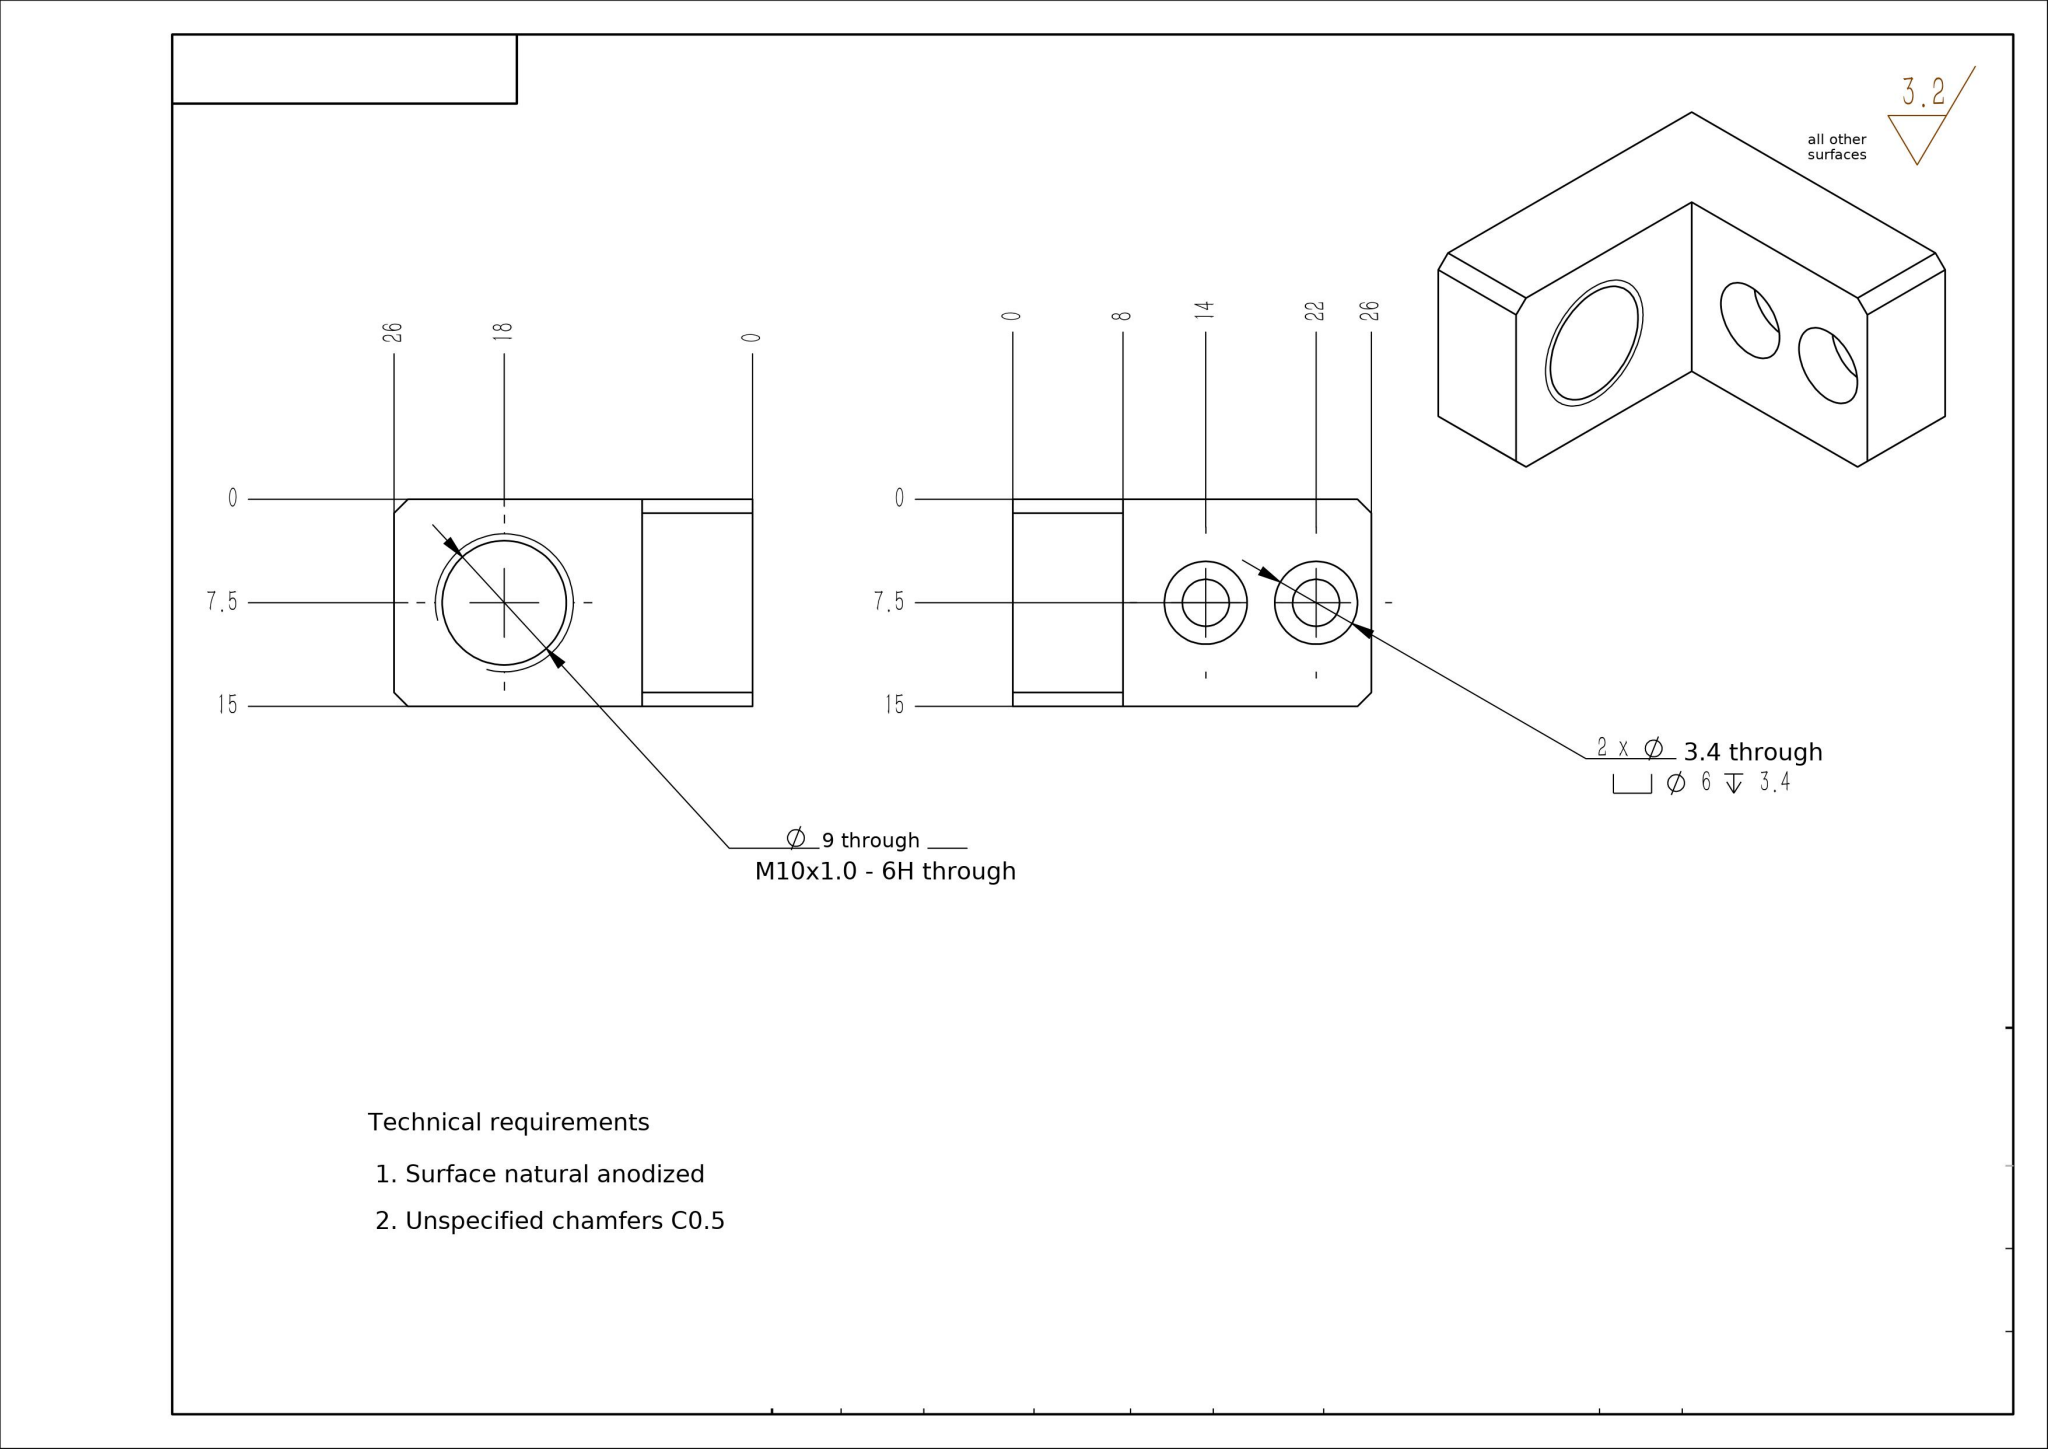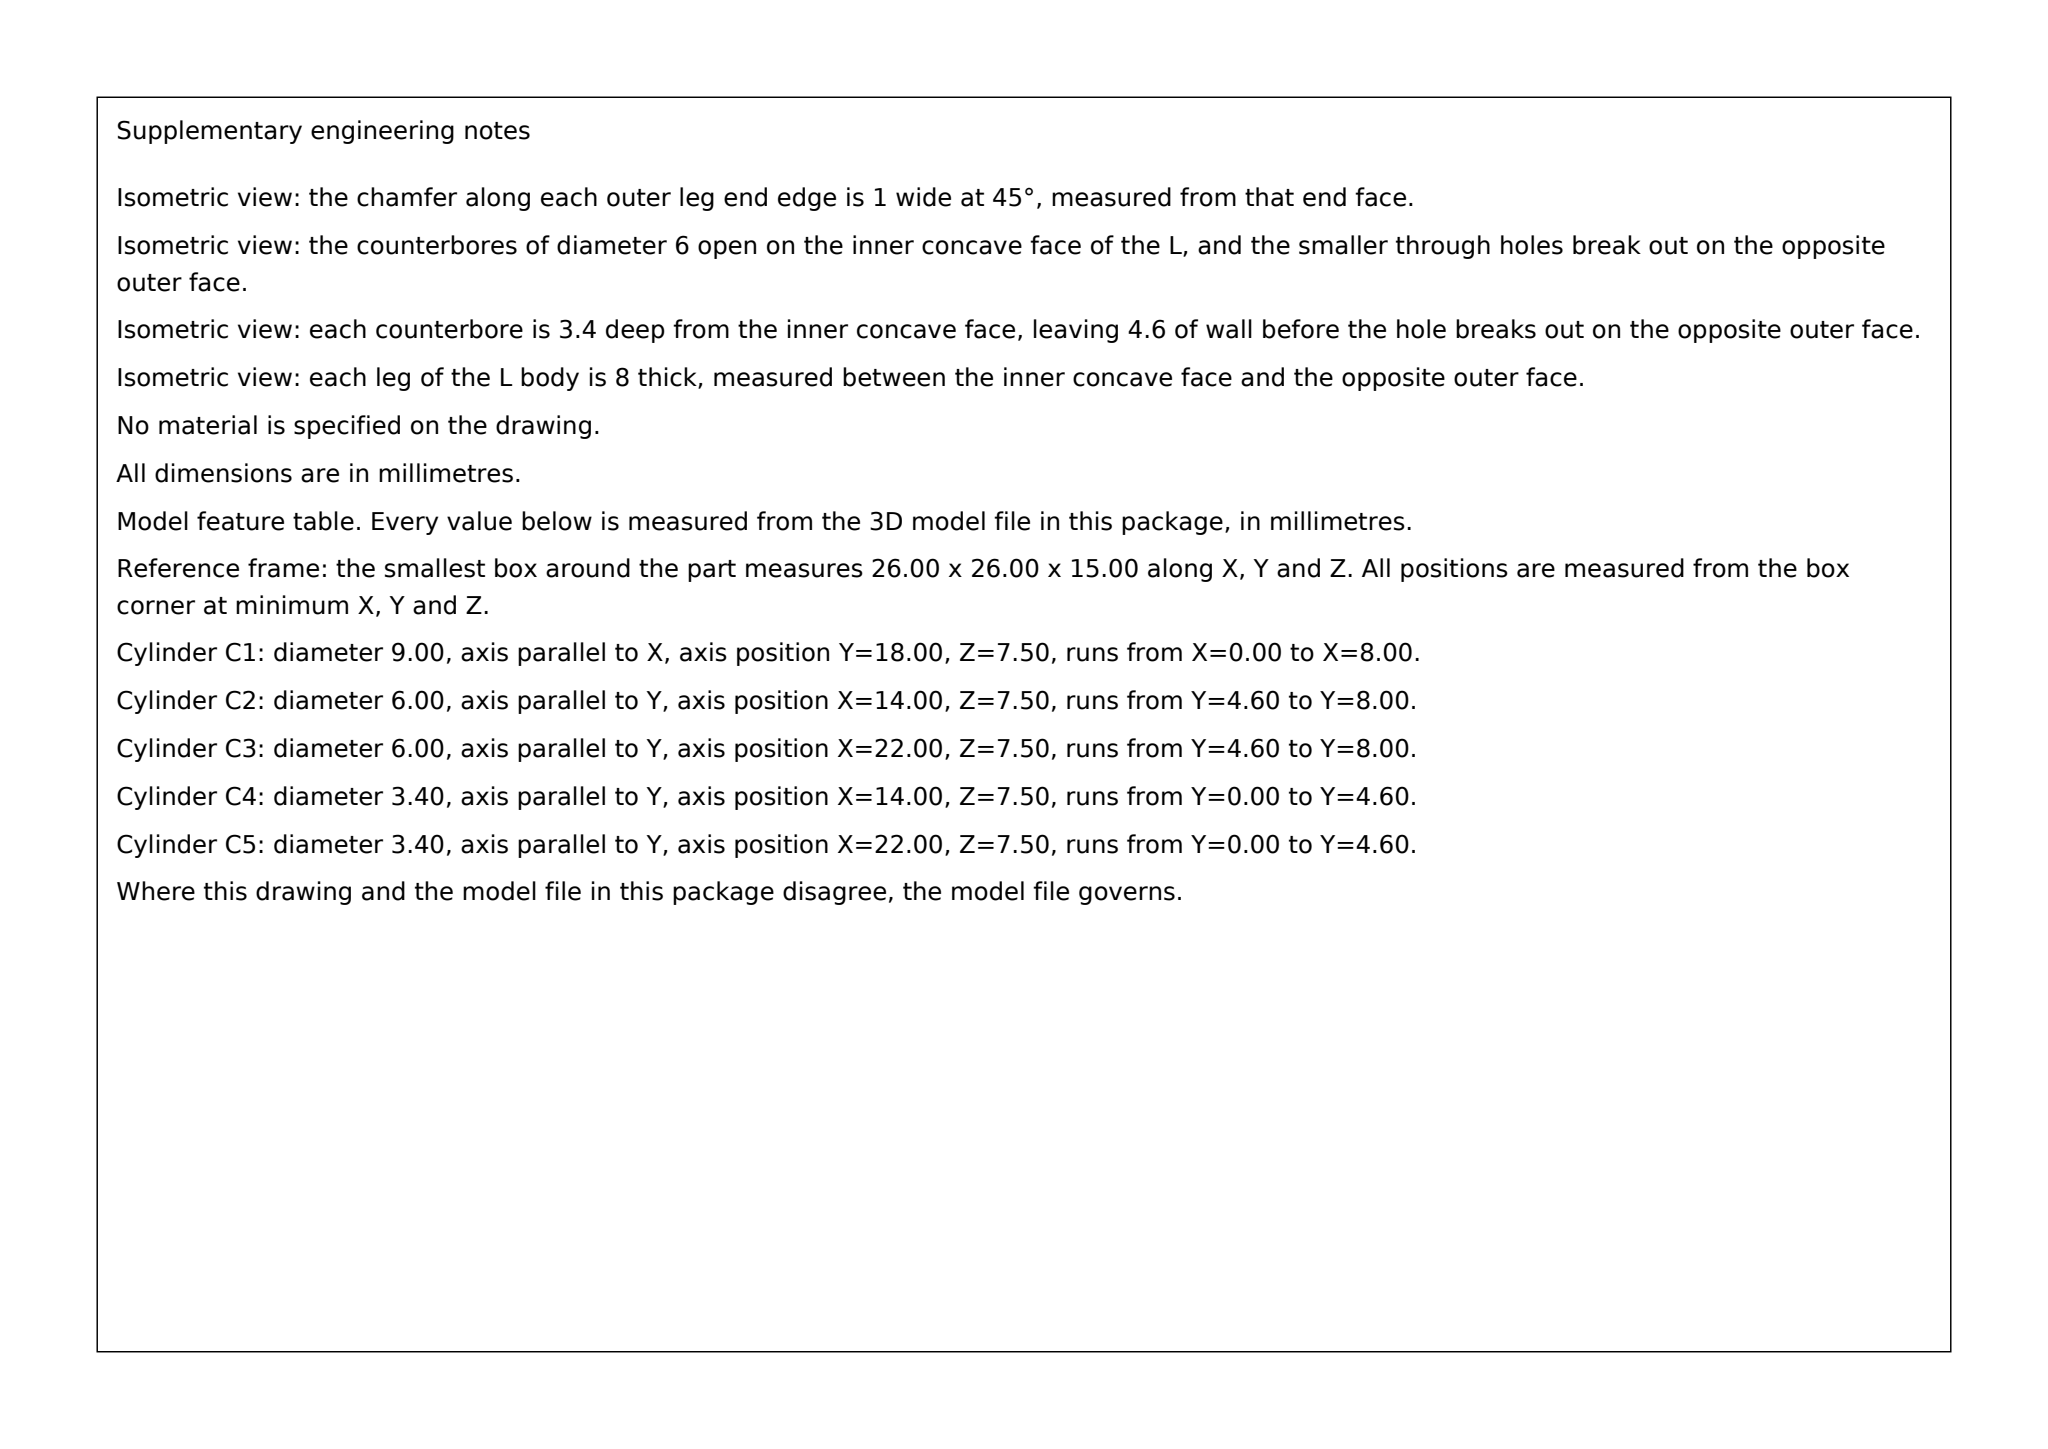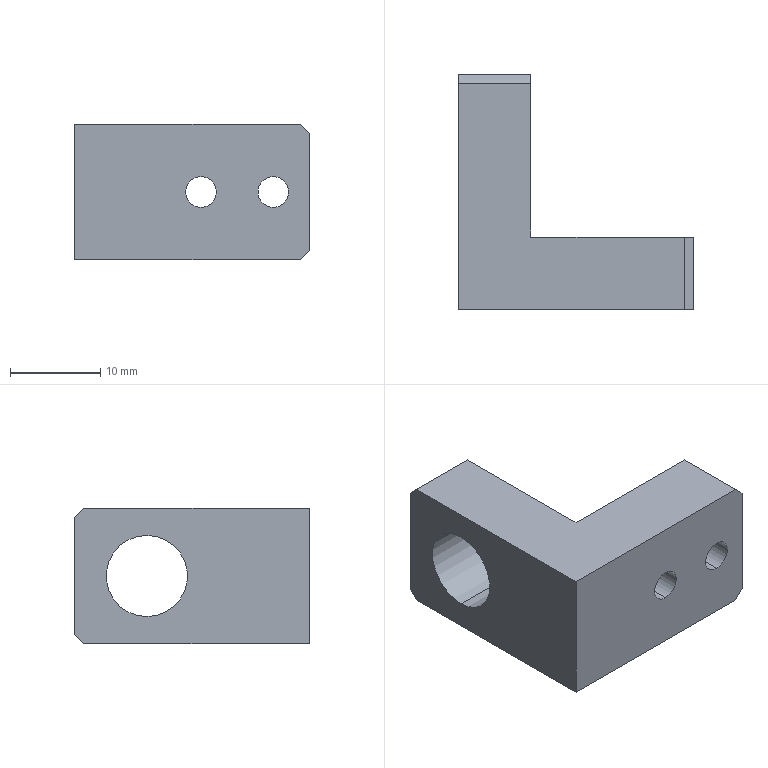Part | SolidWorks | mm | 1 solid | 24 faces | box 26 x 26 x 15 mm | volume 4479 mm3 | plane 14 | cylinder 10 | commonest cylinder face diameters 6 x4 3.4 x4 9 x2
Drawing notes:
LEG THK 8: STEP FACE AT ORD 8 FROM 0 DATUM, BOTH LEGS | from the solid: Planar face y=8 over x 8-26, z 0-15; face x=8 over y 8-26 (symmetric legs, bbox 26x26x15)
4X C1 x 45 ON OUTER CORNER EDGES, 8 LG (NOT C0.5) | from the solid: 4 inclined planes at 45 deg, size 1 x 8 x 1, at x=25/y=25 with z=0 and z=14
M10x1.0-6H THRU 8; Ø9 DRILL THRU | from the solid: Ø9 cylinder, axis x, at y=18 z=7.5, from x=0 to x=8 (full leg thk)
build123d program:
from build123d import *

# Parameters (mm, degrees)
BOSS_EXTRUDE1_DEPTH                               = 15
HOLE_SIZE_ACCORDING_TO_HEXAGON_SOCKET_D           = 3.4
HOLE_SIZE_ACCORDING_TO_HEXAGON_SOCKET_CBORE_D     = 6
HOLE_SIZE_ACCORDING_TO_HEXAGON_SOCKET_CBORE_DEPTH = 3.4
M10X1_0_TAPPED_HOLE1_D                            = 9
CHAMFER1_SIZE                                     = 1
CHAMFER2_SIZE                                     = 1


with BuildPart() as part:
    # Sketch1 → Boss-Extrude1 (new body)
    with BuildSketch(Plane.XY):
        Polygon((-13.935, 19.774), (-13.935, -6.226), (12.065, -6.226), (12.065, 1.774), (-5.935, 1.774), (-5.935, 19.774), align=None)
    extrude(amount=BOSS_EXTRUDE1_DEPTH)

    # Hole Size _ according to_ Hexagon Socket (through all)
    with Locations(Plane(origin=(0, 1.774, 0), x_dir=(1, 0, 0), z_dir=(0, 1, 0))):
        with Locations((8.065, -7.5), (0.06452, -7.5)):
            CounterBoreHole(HOLE_SIZE_ACCORDING_TO_HEXAGON_SOCKET_D / 2, HOLE_SIZE_ACCORDING_TO_HEXAGON_SOCKET_CBORE_D / 2, HOLE_SIZE_ACCORDING_TO_HEXAGON_SOCKET_CBORE_DEPTH)

    # M10x1.0 Tapped Hole1 (through all)
    with Locations(Plane(origin=(-5.935, 0, 0), x_dir=(0, 0, -1), z_dir=(1, 0, 0))):
        with Locations((-7.5, 11.774)):
            Hole(M10X1_0_TAPPED_HOLE1_D / 2)

    # Chamfer1
    chamfer1_edges = [part.edges().sort_by_distance(p)[0] for p in [
        (12.065, -2.226, 15),
        (12.065, -2.226, 0),
    ]]
    chamfer(chamfer1_edges, length=CHAMFER1_SIZE)

    # Chamfer2
    chamfer2_edges = [part.edges().sort_by_distance(p)[0] for p in [
        (-9.935, 19.774, 15),
        (-9.935, 19.774, 0),
    ]]
    chamfer(chamfer2_edges, length=CHAMFER2_SIZE)


solid = part.part
STEP:
#1=CARTESIAN_POINT('',(-13.935,11.774,12.));
#2=VERTEX_POINT('',#1);
#3=CARTESIAN_POINT('',(-13.935,11.774,3.));
#4=VERTEX_POINT('',#3);
#5=CARTESIAN_POINT('',(-13.935,11.774,7.5));
#6=DIRECTION('',(1.,0.,0.));
#7=DIRECTION('',(0.,0.,-1.));
#8=AXIS2_PLACEMENT_3D('',#5,#6,#7);
#9=CIRCLE('',#8,4.5);
#10=EDGE_CURVE('',#2,#4,#9,.T.);
#11=ORIENTED_EDGE('',*,*,#10,.F.);
#12=CARTESIAN_POINT('',(-5.935,11.774,12.));
#13=VERTEX_POINT('',#12);
#14=CARTESIAN_POINT('',(-5.935,11.774,12.));
#15=DIRECTION('',(1.,0.,0.));
#16=VECTOR('',#15,1000.);
#17=LINE('',#14,#16);
#18=EDGE_CURVE('',#2,#13,#17,.T.);
#19=ORIENTED_EDGE('',*,*,#18,.T.);
#20=CARTESIAN_POINT('',(-5.935,11.774,3.));
#21=VERTEX_POINT('',#20);
#22=CARTESIAN_POINT('',(-5.935,11.774,7.5));
#23=DIRECTION('',(1.,0.,0.));
#24=DIRECTION('',(0.,0.,-1.));
#25=AXIS2_PLACEMENT_3D('',#22,#23,#24);
#26=CIRCLE('',#25,4.5);
#27=EDGE_CURVE('',#13,#21,#26,.T.);
#28=ORIENTED_EDGE('',*,*,#27,.T.);
#29=CARTESIAN_POINT('',(-5.935,11.774,3.));
#30=DIRECTION('',(1.,0.,0.));
#31=VECTOR('',#30,1000.);
#32=LINE('',#29,#31);
#33=EDGE_CURVE('',#4,#21,#32,.T.);
#34=ORIENTED_EDGE('',*,*,#33,.F.);
#35=EDGE_LOOP('',(#11,#19,#28,#34));
#36=FACE_OUTER_BOUND('',#35,.T.);
#37=CARTESIAN_POINT('',(-5.935,11.774,7.5));
#38=DIRECTION('',(1.,0.,0.));
#39=DIRECTION('',(0.,0.,-1.));
#40=AXIS2_PLACEMENT_3D('',#37,#38,#39);
#41=CYLINDRICAL_SURFACE('',#40,4.5);
#42=ADVANCED_FACE('',(#36),#41,.F.);
#43=CARTESIAN_POINT('',(8.065,-1.626,4.5));
#44=VERTEX_POINT('',#43);
#45=CARTESIAN_POINT('',(8.065,-1.626,10.5));
#46=VERTEX_POINT('',#45);
#47=CARTESIAN_POINT('',(8.065,-1.626,7.5));
#48=DIRECTION('',(0.,1.,0.));
#49=DIRECTION('',(0.,0.,1.));
#50=AXIS2_PLACEMENT_3D('',#47,#48,#49);
#51=CIRCLE('',#50,3.);
#52=EDGE_CURVE('',#44,#46,#51,.T.);
#53=ORIENTED_EDGE('',*,*,#52,.F.);
#54=CARTESIAN_POINT('',(8.065,1.774,4.5));
#55=VERTEX_POINT('',#54);
#56=CARTESIAN_POINT('',(8.065,1.774,4.5));
#57=DIRECTION('',(0.,1.,0.));
#58=VECTOR('',#57,1000.);
#59=LINE('',#56,#58);
#60=EDGE_CURVE('',#44,#55,#59,.T.);
#61=ORIENTED_EDGE('',*,*,#60,.T.);
#62=CARTESIAN_POINT('',(8.065,1.774,10.5));
#63=VERTEX_POINT('',#62);
#64=CARTESIAN_POINT('',(8.065,1.774,7.5));
#65=DIRECTION('',(0.,1.,0.));
#66=DIRECTION('',(0.,0.,1.));
#67=AXIS2_PLACEMENT_3D('',#64,#65,#66);
#68=CIRCLE('',#67,3.);
#69=EDGE_CURVE('',#55,#63,#68,.T.);
#70=ORIENTED_EDGE('',*,*,#69,.T.);
#71=CARTESIAN_POINT('',(8.065,1.774,10.5));
#72=DIRECTION('',(0.,1.,0.));
#73=VECTOR('',#72,1000.);
#74=LINE('',#71,#73);
#75=EDGE_CURVE('',#46,#63,#74,.T.);
#76=ORIENTED_EDGE('',*,*,#75,.F.);
#77=EDGE_LOOP('',(#53,#61,#70,#76));
#78=FACE_OUTER_BOUND('',#77,.T.);
#79=CARTESIAN_POINT('',(8.065,1.774,7.5));
#80=DIRECTION('',(0.,1.,0.));
#81=DIRECTION('',(0.,0.,1.));
#82=AXIS2_PLACEMENT_3D('',#79,#80,#81);
#83=CYLINDRICAL_SURFACE('',#82,3.);
#84=ADVANCED_FACE('',(#78),#83,.F.);
#85=CARTESIAN_POINT('',(8.065,-6.226,5.8));
#86=VERTEX_POINT('',#85);
#87=CARTESIAN_POINT('',(8.065,-6.226,9.2));
#88=VERTEX_POINT('',#87);
#89=CARTESIAN_POINT('',(8.065,-6.226,7.5));
#90=DIRECTION('',(0.,1.,0.));
#91=DIRECTION('',(0.,0.,1.));
#92=AXIS2_PLACEMENT_3D('',#89,#90,#91);
#93=CIRCLE('',#92,1.7);
#94=EDGE_CURVE('',#86,#88,#93,.T.);
#95=ORIENTED_EDGE('',*,*,#94,.F.);
#96=CARTESIAN_POINT('',(8.065,-1.626,5.8));
#97=VERTEX_POINT('',#96);
#98=CARTESIAN_POINT('',(8.065,1.774,5.8));
#99=DIRECTION('',(0.,1.,0.));
#100=VECTOR('',#99,1000.);
#101=LINE('',#98,#100);
#102=EDGE_CURVE('',#86,#97,#101,.T.);
#103=ORIENTED_EDGE('',*,*,#102,.T.);
#104=CARTESIAN_POINT('',(8.065,-1.626,9.2));
#105=VERTEX_POINT('',#104);
#106=CARTESIAN_POINT('',(8.065,-1.626,7.5));
#107=DIRECTION('',(0.,1.,0.));
#108=DIRECTION('',(0.,0.,1.));
#109=AXIS2_PLACEMENT_3D('',#106,#107,#108);
#110=CIRCLE('',#109,1.7);
#111=EDGE_CURVE('',#97,#105,#110,.T.);
#112=ORIENTED_EDGE('',*,*,#111,.T.);
#113=CARTESIAN_POINT('',(8.065,1.774,9.2));
#114=DIRECTION('',(0.,1.,0.));
#115=VECTOR('',#114,1000.);
#116=LINE('',#113,#115);
#117=EDGE_CURVE('',#88,#105,#116,.T.);
#118=ORIENTED_EDGE('',*,*,#117,.F.);
#119=EDGE_LOOP('',(#95,#103,#112,#118));
#120=FACE_OUTER_BOUND('',#119,.T.);
#121=CARTESIAN_POINT('',(8.065,1.774,7.5));
#122=DIRECTION('',(0.,1.,0.));
#123=DIRECTION('',(0.,0.,1.));
#124=AXIS2_PLACEMENT_3D('',#121,#122,#123);
#125=CYLINDRICAL_SURFACE('',#124,1.7);
#126=ADVANCED_FACE('',(#120),#125,.F.);
#127=CARTESIAN_POINT('',(0.06452,-1.626,4.5));
#128=VERTEX_POINT('',#127);
#129=CARTESIAN_POINT('',(0.06452,-1.626,10.5));
#130=VERTEX_POINT('',#129);
#131=CARTESIAN_POINT('',(0.06452,-1.626,7.5));
#132=DIRECTION('',(0.,1.,0.));
#133=DIRECTION('',(0.,0.,1.));
#134=AXIS2_PLACEMENT_3D('',#131,#132,#133);
#135=CIRCLE('',#134,3.);
#136=EDGE_CURVE('',#128,#130,#135,.T.);
#137=ORIENTED_EDGE('',*,*,#136,.F.);
#138=CARTESIAN_POINT('',(0.06452,1.774,4.5));
#139=VERTEX_POINT('',#138);
#140=CARTESIAN_POINT('',(0.06452,1.774,4.5));
#141=DIRECTION('',(0.,1.,0.));
#142=VECTOR('',#141,1000.);
#143=LINE('',#140,#142);
#144=EDGE_CURVE('',#128,#139,#143,.T.);
#145=ORIENTED_EDGE('',*,*,#144,.T.);
#146=CARTESIAN_POINT('',(0.06452,1.774,10.5));
#147=VERTEX_POINT('',#146);
#148=CARTESIAN_POINT('',(0.06452,1.774,7.5));
#149=DIRECTION('',(0.,1.,0.));
#150=DIRECTION('',(0.,0.,1.));
#151=AXIS2_PLACEMENT_3D('',#148,#149,#150);
#152=CIRCLE('',#151,3.);
#153=EDGE_CURVE('',#139,#147,#152,.T.);
#154=ORIENTED_EDGE('',*,*,#153,.T.);
#155=CARTESIAN_POINT('',(0.06452,1.774,10.5));
#156=DIRECTION('',(0.,1.,0.));
#157=VECTOR('',#156,1000.);
#158=LINE('',#155,#157);
#159=EDGE_CURVE('',#130,#147,#158,.T.);
#160=ORIENTED_EDGE('',*,*,#159,.F.);
#161=EDGE_LOOP('',(#137,#145,#154,#160));
#162=FACE_OUTER_BOUND('',#161,.T.);
#163=CARTESIAN_POINT('',(0.06452,1.774,7.5));
#164=DIRECTION('',(0.,1.,0.));
#165=DIRECTION('',(0.,0.,1.));
#166=AXIS2_PLACEMENT_3D('',#163,#164,#165);
#167=CYLINDRICAL_SURFACE('',#166,3.);
#168=ADVANCED_FACE('',(#162),#167,.F.);
#169=CARTESIAN_POINT('',(0.06452,-6.226,5.8));
#170=VERTEX_POINT('',#169);
#171=CARTESIAN_POINT('',(0.06452,-6.226,9.2));
#172=VERTEX_POINT('',#171);
#173=CARTESIAN_POINT('',(0.06452,-6.226,7.5));
#174=DIRECTION('',(0.,1.,0.));
#175=DIRECTION('',(0.,0.,1.));
#176=AXIS2_PLACEMENT_3D('',#173,#174,#175);
#177=CIRCLE('',#176,1.7);
#178=EDGE_CURVE('',#170,#172,#177,.T.);
#179=ORIENTED_EDGE('',*,*,#178,.F.);
#180=CARTESIAN_POINT('',(0.06452,-1.626,5.8));
#181=VERTEX_POINT('',#180);
#182=CARTESIAN_POINT('',(0.06452,1.774,5.8));
#183=DIRECTION('',(0.,1.,0.));
#184=VECTOR('',#183,1000.);
#185=LINE('',#182,#184);
#186=EDGE_CURVE('',#170,#181,#185,.T.);
#187=ORIENTED_EDGE('',*,*,#186,.T.);
#188=CARTESIAN_POINT('',(0.06452,-1.626,9.2));
#189=VERTEX_POINT('',#188);
#190=CARTESIAN_POINT('',(0.06452,-1.626,7.5));
#191=DIRECTION('',(0.,1.,0.));
#192=DIRECTION('',(0.,0.,1.));
#193=AXIS2_PLACEMENT_3D('',#190,#191,#192);
#194=CIRCLE('',#193,1.7);
#195=EDGE_CURVE('',#181,#189,#194,.T.);
#196=ORIENTED_EDGE('',*,*,#195,.T.);
#197=CARTESIAN_POINT('',(0.06452,1.774,9.2));
#198=DIRECTION('',(0.,1.,0.));
#199=VECTOR('',#198,1000.);
#200=LINE('',#197,#199);
#201=EDGE_CURVE('',#172,#189,#200,.T.);
#202=ORIENTED_EDGE('',*,*,#201,.F.);
#203=EDGE_LOOP('',(#179,#187,#196,#202));
#204=FACE_OUTER_BOUND('',#203,.T.);
#205=CARTESIAN_POINT('',(0.06452,1.774,7.5));
#206=DIRECTION('',(0.,1.,0.));
#207=DIRECTION('',(0.,0.,1.));
#208=AXIS2_PLACEMENT_3D('',#205,#206,#207);
#209=CYLINDRICAL_SURFACE('',#208,1.7);
#210=ADVANCED_FACE('',(#204),#209,.F.);
#211=CARTESIAN_POINT('',(-5.935,19.774,14.));
#212=VERTEX_POINT('',#211);
#213=CARTESIAN_POINT('',(-5.935,19.774,1.));
#214=VERTEX_POINT('',#213);
#215=CARTESIAN_POINT('',(-5.935,19.774,15.));
#216=DIRECTION('',(0.,0.,-1.));
#217=VECTOR('',#216,1000.);
#218=LINE('',#215,#217);
#219=EDGE_CURVE('',#212,#214,#218,.T.);
#220=ORIENTED_EDGE('',*,*,#219,.T.);
#221=CARTESIAN_POINT('',(-13.935,19.774,1.));
#222=VERTEX_POINT('',#221);
#223=CARTESIAN_POINT('',(-5.935,19.774,1.));
#224=DIRECTION('',(-1.,0.,0.));
#225=VECTOR('',#224,1000.);
#226=LINE('',#223,#225);
#227=EDGE_CURVE('',#214,#222,#226,.T.);
#228=ORIENTED_EDGE('',*,*,#227,.T.);
#229=CARTESIAN_POINT('',(-13.935,19.774,14.));
#230=VERTEX_POINT('',#229);
#231=CARTESIAN_POINT('',(-13.935,19.774,15.));
#232=DIRECTION('',(0.,0.,-1.));
#233=VECTOR('',#232,1000.);
#234=LINE('',#231,#233);
#235=EDGE_CURVE('',#230,#222,#234,.T.);
#236=ORIENTED_EDGE('',*,*,#235,.F.);
#237=CARTESIAN_POINT('',(-5.935,19.774,14.));
#238=DIRECTION('',(1.,0.,0.));
#239=VECTOR('',#238,1000.);
#240=LINE('',#237,#239);
#241=EDGE_CURVE('',#230,#212,#240,.T.);
#242=ORIENTED_EDGE('',*,*,#241,.T.);
#243=EDGE_LOOP('',(#220,#228,#236,#242));
#244=FACE_OUTER_BOUND('',#243,.T.);
#245=CARTESIAN_POINT('',(-5.935,19.774,15.));
#246=DIRECTION('',(0.,-1.,0.));
#247=DIRECTION('',(0.,0.,-1.));
#248=AXIS2_PLACEMENT_3D('',#245,#246,#247);
#249=PLANE('',#248);
#250=ADVANCED_FACE('',(#244),#249,.F.);
#251=CARTESIAN_POINT('',(-13.935,11.774,7.5));
#252=DIRECTION('',(1.,0.,0.));
#253=DIRECTION('',(0.,0.,-1.));
#254=AXIS2_PLACEMENT_3D('',#251,#252,#253);
#255=CIRCLE('',#254,4.5);
#256=EDGE_CURVE('',#4,#2,#255,.T.);
#257=ORIENTED_EDGE('',*,*,#256,.T.);
#258=ORIENTED_EDGE('',*,*,#10,.T.);
#259=EDGE_LOOP('',(#257,#258));
#260=FACE_BOUND('',#259,.T.);
#261=ORIENTED_EDGE('',*,*,#235,.T.);
#262=CARTESIAN_POINT('',(-13.935,18.774,0.));
#263=VERTEX_POINT('',#262);
#264=CARTESIAN_POINT('',(-13.935,19.774,1.));
#265=DIRECTION('',(0.,-0.7071,-0.7071));
#266=VECTOR('',#265,1000.);
#267=LINE('',#264,#266);
#268=EDGE_CURVE('',#222,#263,#267,.T.);
#269=ORIENTED_EDGE('',*,*,#268,.T.);
#270=CARTESIAN_POINT('',(-13.935,-6.226,0.));
#271=VERTEX_POINT('',#270);
#272=CARTESIAN_POINT('',(-13.935,19.774,0.));
#273=DIRECTION('',(0.,-1.,0.));
#274=VECTOR('',#273,1000.);
#275=LINE('',#272,#274);
#276=EDGE_CURVE('',#263,#271,#275,.T.);
#277=ORIENTED_EDGE('',*,*,#276,.T.);
#278=CARTESIAN_POINT('',(-13.935,-6.226,15.));
#279=VERTEX_POINT('',#278);
#280=CARTESIAN_POINT('',(-13.935,-6.226,15.));
#281=DIRECTION('',(0.,0.,-1.));
#282=VECTOR('',#281,1000.);
#283=LINE('',#280,#282);
#284=EDGE_CURVE('',#279,#271,#283,.T.);
#285=ORIENTED_EDGE('',*,*,#284,.F.);
#286=CARTESIAN_POINT('',(-13.935,18.774,15.));
#287=VERTEX_POINT('',#286);
#288=CARTESIAN_POINT('',(-13.935,19.774,15.));
#289=DIRECTION('',(0.,-1.,0.));
#290=VECTOR('',#289,1000.);
#291=LINE('',#288,#290);
#292=EDGE_CURVE('',#287,#279,#291,.T.);
#293=ORIENTED_EDGE('',*,*,#292,.F.);
#294=CARTESIAN_POINT('',(-13.935,18.774,15.));
#295=DIRECTION('',(-0.,0.7071,-0.7071));
#296=VECTOR('',#295,1000.);
#297=LINE('',#294,#296);
#298=EDGE_CURVE('',#287,#230,#297,.T.);
#299=ORIENTED_EDGE('',*,*,#298,.T.);
#300=EDGE_LOOP('',(#261,#269,#277,#285,#293,#299));
#301=FACE_OUTER_BOUND('',#300,.T.);
#302=CARTESIAN_POINT('',(-13.935,19.774,15.));
#303=DIRECTION('',(1.,0.,0.));
#304=DIRECTION('',(-0.,1.,0.));
#305=AXIS2_PLACEMENT_3D('',#302,#303,#304);
#306=PLANE('',#305);
#307=ADVANCED_FACE('',(#260,#301),#306,.F.);
#308=CARTESIAN_POINT('',(8.065,-6.226,7.5));
#309=DIRECTION('',(0.,1.,0.));
#310=DIRECTION('',(0.,0.,1.));
#311=AXIS2_PLACEMENT_3D('',#308,#309,#310);
#312=CIRCLE('',#311,1.7);
#313=EDGE_CURVE('',#88,#86,#312,.T.);
#314=ORIENTED_EDGE('',*,*,#313,.T.);
#315=ORIENTED_EDGE('',*,*,#94,.T.);
#316=EDGE_LOOP('',(#314,#315));
#317=FACE_BOUND('',#316,.T.);
#318=CARTESIAN_POINT('',(0.06452,-6.226,7.5));
#319=DIRECTION('',(0.,1.,0.));
#320=DIRECTION('',(0.,0.,1.));
#321=AXIS2_PLACEMENT_3D('',#318,#319,#320);
#322=CIRCLE('',#321,1.7);
#323=EDGE_CURVE('',#172,#170,#322,.T.);
#324=ORIENTED_EDGE('',*,*,#323,.T.);
#325=ORIENTED_EDGE('',*,*,#178,.T.);
#326=EDGE_LOOP('',(#324,#325));
#327=FACE_BOUND('',#326,.T.);
#328=CARTESIAN_POINT('',(12.065,-6.226,14.));
#329=VERTEX_POINT('',#328);
#330=CARTESIAN_POINT('',(12.065,-6.226,1.));
#331=VERTEX_POINT('',#330);
#332=CARTESIAN_POINT('',(12.065,-6.226,15.));
#333=DIRECTION('',(0.,0.,-1.));
#334=VECTOR('',#333,1000.);
#335=LINE('',#332,#334);
#336=EDGE_CURVE('',#329,#331,#335,.T.);
#337=ORIENTED_EDGE('',*,*,#336,.F.);
#338=CARTESIAN_POINT('',(11.065,-6.226,15.));
#339=VERTEX_POINT('',#338);
#340=CARTESIAN_POINT('',(11.065,-6.226,15.));
#341=DIRECTION('',(-0.7071,0.,0.7071));
#342=VECTOR('',#341,1000.);
#343=LINE('',#340,#342);
#344=EDGE_CURVE('',#329,#339,#343,.T.);
#345=ORIENTED_EDGE('',*,*,#344,.T.);
#346=CARTESIAN_POINT('',(-13.935,-6.226,15.));
#347=DIRECTION('',(1.,0.,0.));
#348=VECTOR('',#347,1000.);
#349=LINE('',#346,#348);
#350=EDGE_CURVE('',#279,#339,#349,.T.);
#351=ORIENTED_EDGE('',*,*,#350,.F.);
#352=ORIENTED_EDGE('',*,*,#284,.T.);
#353=CARTESIAN_POINT('',(11.065,-6.226,-0.));
#354=VERTEX_POINT('',#353);
#355=CARTESIAN_POINT('',(-13.935,-6.226,0.));
#356=DIRECTION('',(1.,0.,0.));
#357=VECTOR('',#356,1000.);
#358=LINE('',#355,#357);
#359=EDGE_CURVE('',#271,#354,#358,.T.);
#360=ORIENTED_EDGE('',*,*,#359,.T.);
#361=CARTESIAN_POINT('',(12.065,-6.226,1.));
#362=DIRECTION('',(0.7071,0.,0.7071));
#363=VECTOR('',#362,1000.);
#364=LINE('',#361,#363);
#365=EDGE_CURVE('',#354,#331,#364,.T.);
#366=ORIENTED_EDGE('',*,*,#365,.T.);
#367=EDGE_LOOP('',(#337,#345,#351,#352,#360,#366));
#368=FACE_OUTER_BOUND('',#367,.T.);
#369=CARTESIAN_POINT('',(-13.935,-6.226,15.));
#370=DIRECTION('',(0.,1.,0.));
#371=DIRECTION('',(0.,0.,1.));
#372=AXIS2_PLACEMENT_3D('',#369,#370,#371);
#373=PLANE('',#372);
#374=ADVANCED_FACE('',(#317,#327,#368),#373,.F.);
#375=CARTESIAN_POINT('',(12.065,1.774,14.));
#376=VERTEX_POINT('',#375);
#377=CARTESIAN_POINT('',(12.065,1.774,1.));
#378=VERTEX_POINT('',#377);
#379=CARTESIAN_POINT('',(12.065,1.774,15.));
#380=DIRECTION('',(0.,0.,-1.));
#381=VECTOR('',#380,1000.);
#382=LINE('',#379,#381);
#383=EDGE_CURVE('',#376,#378,#382,.T.);
#384=ORIENTED_EDGE('',*,*,#383,.F.);
#385=CARTESIAN_POINT('',(12.065,-6.226,14.));
#386=DIRECTION('',(0.,-1.,0.));
#387=VECTOR('',#386,1000.);
#388=LINE('',#385,#387);
#389=EDGE_CURVE('',#376,#329,#388,.T.);
#390=ORIENTED_EDGE('',*,*,#389,.T.);
#391=ORIENTED_EDGE('',*,*,#336,.T.);
#392=CARTESIAN_POINT('',(12.065,-6.226,1.));
#393=DIRECTION('',(0.,1.,0.));
#394=VECTOR('',#393,1000.);
#395=LINE('',#392,#394);
#396=EDGE_CURVE('',#331,#378,#395,.T.);
#397=ORIENTED_EDGE('',*,*,#396,.T.);
#398=EDGE_LOOP('',(#384,#390,#391,#397));
#399=FACE_OUTER_BOUND('',#398,.T.);
#400=CARTESIAN_POINT('',(12.065,-6.226,15.));
#401=DIRECTION('',(-1.,0.,0.));
#402=DIRECTION('',(0.,0.,1.));
#403=AXIS2_PLACEMENT_3D('',#400,#401,#402);
#404=PLANE('',#403);
#405=ADVANCED_FACE('',(#399),#404,.F.);
#406=CARTESIAN_POINT('',(8.065,1.774,7.5));
#407=DIRECTION('',(0.,1.,0.));
#408=DIRECTION('',(0.,0.,1.));
#409=AXIS2_PLACEMENT_3D('',#406,#407,#408);
#410=CIRCLE('',#409,3.);
#411=EDGE_CURVE('',#63,#55,#410,.T.);
#412=ORIENTED_EDGE('',*,*,#411,.F.);
#413=ORIENTED_EDGE('',*,*,#69,.F.);
#414=EDGE_LOOP('',(#412,#413));
#415=FACE_BOUND('',#414,.T.);
#416=CARTESIAN_POINT('',(0.06452,1.774,7.5));
#417=DIRECTION('',(0.,1.,0.));
#418=DIRECTION('',(0.,0.,1.));
#419=AXIS2_PLACEMENT_3D('',#416,#417,#418);
#420=CIRCLE('',#419,3.);
#421=EDGE_CURVE('',#147,#139,#420,.T.);
#422=ORIENTED_EDGE('',*,*,#421,.F.);
#423=ORIENTED_EDGE('',*,*,#153,.F.);
#424=EDGE_LOOP('',(#422,#423));
#425=FACE_BOUND('',#424,.T.);
#426=CARTESIAN_POINT('',(11.065,1.774,15.));
#427=VERTEX_POINT('',#426);
#428=CARTESIAN_POINT('',(-5.935,1.774,15.));
#429=VERTEX_POINT('',#428);
#430=CARTESIAN_POINT('',(12.065,1.774,15.));
#431=DIRECTION('',(-1.,-0.,0.));
#432=VECTOR('',#431,1000.);
#433=LINE('',#430,#432);
#434=EDGE_CURVE('',#427,#429,#433,.T.);
#435=ORIENTED_EDGE('',*,*,#434,.F.);
#436=CARTESIAN_POINT('',(11.065,1.774,15.));
#437=DIRECTION('',(0.7071,0.,-0.7071));
#438=VECTOR('',#437,1000.);
#439=LINE('',#436,#438);
#440=EDGE_CURVE('',#427,#376,#439,.T.);
#441=ORIENTED_EDGE('',*,*,#440,.T.);
#442=ORIENTED_EDGE('',*,*,#383,.T.);
#443=CARTESIAN_POINT('',(11.065,1.774,0.));
#444=VERTEX_POINT('',#443);
#445=CARTESIAN_POINT('',(12.065,1.774,1.));
#446=DIRECTION('',(-0.7071,-0.,-0.7071));
#447=VECTOR('',#446,1000.);
#448=LINE('',#445,#447);
#449=EDGE_CURVE('',#378,#444,#448,.T.);
#450=ORIENTED_EDGE('',*,*,#449,.T.);
#451=CARTESIAN_POINT('',(-5.935,1.774,0.));
#452=VERTEX_POINT('',#451);
#453=CARTESIAN_POINT('',(12.065,1.774,0.));
#454=DIRECTION('',(-1.,-0.,0.));
#455=VECTOR('',#454,1000.);
#456=LINE('',#453,#455);
#457=EDGE_CURVE('',#444,#452,#456,.T.);
#458=ORIENTED_EDGE('',*,*,#457,.T.);
#459=CARTESIAN_POINT('',(-5.935,1.774,15.));
#460=DIRECTION('',(0.,0.,-1.));
#461=VECTOR('',#460,1000.);
#462=LINE('',#459,#461);
#463=EDGE_CURVE('',#429,#452,#462,.T.);
#464=ORIENTED_EDGE('',*,*,#463,.F.);
#465=EDGE_LOOP('',(#435,#441,#442,#450,#458,#464));
#466=FACE_OUTER_BOUND('',#465,.T.);
#467=CARTESIAN_POINT('',(12.065,1.774,15.));
#468=DIRECTION('',(0.,-1.,0.));
#469=DIRECTION('',(1.,0.,0.));
#470=AXIS2_PLACEMENT_3D('',#467,#468,#469);
#471=PLANE('',#470);
#472=ADVANCED_FACE('',(#415,#425,#466),#471,.F.);
#473=CARTESIAN_POINT('',(-5.935,11.774,7.5));
#474=DIRECTION('',(1.,0.,0.));
#475=DIRECTION('',(0.,0.,-1.));
#476=AXIS2_PLACEMENT_3D('',#473,#474,#475);
#477=CIRCLE('',#476,4.5);
#478=EDGE_CURVE('',#21,#13,#477,.T.);
#479=ORIENTED_EDGE('',*,*,#478,.F.);
#480=ORIENTED_EDGE('',*,*,#27,.F.);
#481=EDGE_LOOP('',(#479,#480));
#482=FACE_BOUND('',#481,.T.);
#483=CARTESIAN_POINT('',(-5.935,18.774,0.));
#484=VERTEX_POINT('',#483);
#485=CARTESIAN_POINT('',(-5.935,1.774,0.));
#486=DIRECTION('',(0.,1.,0.));
#487=VECTOR('',#486,1000.);
#488=LINE('',#485,#487);
#489=EDGE_CURVE('',#452,#484,#488,.T.);
#490=ORIENTED_EDGE('',*,*,#489,.T.);
#491=CARTESIAN_POINT('',(-5.935,19.774,1.));
#492=DIRECTION('',(0.,0.7071,0.7071));
#493=VECTOR('',#492,1000.);
#494=LINE('',#491,#493);
#495=EDGE_CURVE('',#484,#214,#494,.T.);
#496=ORIENTED_EDGE('',*,*,#495,.T.);
#497=ORIENTED_EDGE('',*,*,#219,.F.);
#498=CARTESIAN_POINT('',(-5.935,18.774,15.));
#499=VERTEX_POINT('',#498);
#500=CARTESIAN_POINT('',(-5.935,18.774,15.));
#501=DIRECTION('',(-0.,-0.7071,0.7071));
#502=VECTOR('',#501,1000.);
#503=LINE('',#500,#502);
#504=EDGE_CURVE('',#212,#499,#503,.T.);
#505=ORIENTED_EDGE('',*,*,#504,.T.);
#506=CARTESIAN_POINT('',(-5.935,1.774,15.));
#507=DIRECTION('',(0.,1.,0.));
#508=VECTOR('',#507,1000.);
#509=LINE('',#506,#508);
#510=EDGE_CURVE('',#429,#499,#509,.T.);
#511=ORIENTED_EDGE('',*,*,#510,.F.);
#512=ORIENTED_EDGE('',*,*,#463,.T.);
#513=EDGE_LOOP('',(#490,#496,#497,#505,#511,#512));
#514=FACE_OUTER_BOUND('',#513,.T.);
#515=CARTESIAN_POINT('',(-5.935,1.774,15.));
#516=DIRECTION('',(-1.,0.,0.));
#517=DIRECTION('',(-0.,-1.,0.));
#518=AXIS2_PLACEMENT_3D('',#515,#516,#517);
#519=PLANE('',#518);
#520=ADVANCED_FACE('',(#482,#514),#519,.F.);
#521=ORIENTED_EDGE('',*,*,#510,.T.);
#522=CARTESIAN_POINT('',(-13.935,18.774,15.));
#523=DIRECTION('',(-1.,0.,0.));
#524=VECTOR('',#523,1000.);
#525=LINE('',#522,#524);
#526=EDGE_CURVE('',#499,#287,#525,.T.);
#527=ORIENTED_EDGE('',*,*,#526,.T.);
#528=ORIENTED_EDGE('',*,*,#292,.T.);
#529=ORIENTED_EDGE('',*,*,#350,.T.);
#530=CARTESIAN_POINT('',(11.065,1.774,15.));
#531=DIRECTION('',(0.,1.,0.));
#532=VECTOR('',#531,1000.);
#533=LINE('',#530,#532);
#534=EDGE_CURVE('',#339,#427,#533,.T.);
#535=ORIENTED_EDGE('',*,*,#534,.T.);
#536=ORIENTED_EDGE('',*,*,#434,.T.);
#537=EDGE_LOOP('',(#521,#527,#528,#529,#535,#536));
#538=FACE_OUTER_BOUND('',#537,.T.);
#539=CARTESIAN_POINT('',(0.,0.,15.));
#540=DIRECTION('',(0.,0.,1.));
#541=DIRECTION('',(1.,0.,0.));
#542=AXIS2_PLACEMENT_3D('',#539,#540,#541);
#543=PLANE('',#542);
#544=ADVANCED_FACE('',(#538),#543,.T.);
#545=ORIENTED_EDGE('',*,*,#276,.F.);
#546=CARTESIAN_POINT('',(0.,18.774,0.));
#547=DIRECTION('',(1.,0.,0.));
#548=VECTOR('',#547,1000.);
#549=LINE('',#546,#548);
#550=EDGE_CURVE('',#263,#484,#549,.T.);
#551=ORIENTED_EDGE('',*,*,#550,.T.);
#552=ORIENTED_EDGE('',*,*,#489,.F.);
#553=ORIENTED_EDGE('',*,*,#457,.F.);
#554=CARTESIAN_POINT('',(11.065,0.,0.));
#555=DIRECTION('',(0.,-1.,0.));
#556=VECTOR('',#555,1000.);
#557=LINE('',#554,#556);
#558=EDGE_CURVE('',#444,#354,#557,.T.);
#559=ORIENTED_EDGE('',*,*,#558,.T.);
#560=ORIENTED_EDGE('',*,*,#359,.F.);
#561=EDGE_LOOP('',(#545,#551,#552,#553,#559,#560));
#562=FACE_OUTER_BOUND('',#561,.T.);
#563=CARTESIAN_POINT('',(0.,0.,0.));
#564=DIRECTION('',(0.,0.,1.));
#565=DIRECTION('',(1.,0.,0.));
#566=AXIS2_PLACEMENT_3D('',#563,#564,#565);
#567=PLANE('',#566);
#568=ADVANCED_FACE('',(#562),#567,.F.);
#569=ORIENTED_EDGE('',*,*,#186,.F.);
#570=ORIENTED_EDGE('',*,*,#323,.F.);
#571=ORIENTED_EDGE('',*,*,#201,.T.);
#572=CARTESIAN_POINT('',(0.06452,-1.626,7.5));
#573=DIRECTION('',(0.,1.,0.));
#574=DIRECTION('',(0.,0.,1.));
#575=AXIS2_PLACEMENT_3D('',#572,#573,#574);
#576=CIRCLE('',#575,1.7);
#577=EDGE_CURVE('',#189,#181,#576,.T.);
#578=ORIENTED_EDGE('',*,*,#577,.T.);
#579=EDGE_LOOP('',(#569,#570,#571,#578));
#580=FACE_OUTER_BOUND('',#579,.T.);
#581=CARTESIAN_POINT('',(0.06452,1.774,7.5));
#582=DIRECTION('',(0.,1.,0.));
#583=DIRECTION('',(0.,0.,1.));
#584=AXIS2_PLACEMENT_3D('',#581,#582,#583);
#585=CYLINDRICAL_SURFACE('',#584,1.7);
#586=ADVANCED_FACE('',(#580),#585,.F.);
#587=ORIENTED_EDGE('',*,*,#577,.F.);
#588=ORIENTED_EDGE('',*,*,#195,.F.);
#589=EDGE_LOOP('',(#587,#588));
#590=FACE_BOUND('',#589,.T.);
#591=CARTESIAN_POINT('',(0.06452,-1.626,7.5));
#592=DIRECTION('',(0.,1.,0.));
#593=DIRECTION('',(0.,0.,1.));
#594=AXIS2_PLACEMENT_3D('',#591,#592,#593);
#595=CIRCLE('',#594,3.);
#596=EDGE_CURVE('',#130,#128,#595,.T.);
#597=ORIENTED_EDGE('',*,*,#596,.T.);
#598=ORIENTED_EDGE('',*,*,#136,.T.);
#599=EDGE_LOOP('',(#597,#598));
#600=FACE_OUTER_BOUND('',#599,.T.);
#601=CARTESIAN_POINT('',(1.765,-1.626,7.5));
#602=DIRECTION('',(0.,-1.,0.));
#603=DIRECTION('',(0.,0.,-1.));
#604=AXIS2_PLACEMENT_3D('',#601,#602,#603);
#605=PLANE('',#604);
#606=ADVANCED_FACE('',(#590,#600),#605,.F.);
#607=ORIENTED_EDGE('',*,*,#144,.F.);
#608=ORIENTED_EDGE('',*,*,#596,.F.);
#609=ORIENTED_EDGE('',*,*,#159,.T.);
#610=ORIENTED_EDGE('',*,*,#421,.T.);
#611=EDGE_LOOP('',(#607,#608,#609,#610));
#612=FACE_OUTER_BOUND('',#611,.T.);
#613=CARTESIAN_POINT('',(0.06452,1.774,7.5));
#614=DIRECTION('',(0.,1.,0.));
#615=DIRECTION('',(0.,0.,1.));
#616=AXIS2_PLACEMENT_3D('',#613,#614,#615);
#617=CYLINDRICAL_SURFACE('',#616,3.);
#618=ADVANCED_FACE('',(#612),#617,.F.);
#619=ORIENTED_EDGE('',*,*,#102,.F.);
#620=ORIENTED_EDGE('',*,*,#313,.F.);
#621=ORIENTED_EDGE('',*,*,#117,.T.);
#622=CARTESIAN_POINT('',(8.065,-1.626,7.5));
#623=DIRECTION('',(0.,1.,0.));
#624=DIRECTION('',(0.,0.,1.));
#625=AXIS2_PLACEMENT_3D('',#622,#623,#624);
#626=CIRCLE('',#625,1.7);
#627=EDGE_CURVE('',#105,#97,#626,.T.);
#628=ORIENTED_EDGE('',*,*,#627,.T.);
#629=EDGE_LOOP('',(#619,#620,#621,#628));
#630=FACE_OUTER_BOUND('',#629,.T.);
#631=CARTESIAN_POINT('',(8.065,1.774,7.5));
#632=DIRECTION('',(0.,1.,0.));
#633=DIRECTION('',(0.,0.,1.));
#634=AXIS2_PLACEMENT_3D('',#631,#632,#633);
#635=CYLINDRICAL_SURFACE('',#634,1.7);
#636=ADVANCED_FACE('',(#630),#635,.F.);
#637=ORIENTED_EDGE('',*,*,#627,.F.);
#638=ORIENTED_EDGE('',*,*,#111,.F.);
#639=EDGE_LOOP('',(#637,#638));
#640=FACE_BOUND('',#639,.T.);
#641=CARTESIAN_POINT('',(8.065,-1.626,7.5));
#642=DIRECTION('',(0.,1.,0.));
#643=DIRECTION('',(0.,0.,1.));
#644=AXIS2_PLACEMENT_3D('',#641,#642,#643);
#645=CIRCLE('',#644,3.);
#646=EDGE_CURVE('',#46,#44,#645,.T.);
#647=ORIENTED_EDGE('',*,*,#646,.T.);
#648=ORIENTED_EDGE('',*,*,#52,.T.);
#649=EDGE_LOOP('',(#647,#648));
#650=FACE_OUTER_BOUND('',#649,.T.);
#651=CARTESIAN_POINT('',(9.765,-1.626,7.5));
#652=DIRECTION('',(0.,-1.,0.));
#653=DIRECTION('',(0.,0.,-1.));
#654=AXIS2_PLACEMENT_3D('',#651,#652,#653);
#655=PLANE('',#654);
#656=ADVANCED_FACE('',(#640,#650),#655,.F.);
#657=ORIENTED_EDGE('',*,*,#60,.F.);
#658=ORIENTED_EDGE('',*,*,#646,.F.);
#659=ORIENTED_EDGE('',*,*,#75,.T.);
#660=ORIENTED_EDGE('',*,*,#411,.T.);
#661=EDGE_LOOP('',(#657,#658,#659,#660));
#662=FACE_OUTER_BOUND('',#661,.T.);
#663=CARTESIAN_POINT('',(8.065,1.774,7.5));
#664=DIRECTION('',(0.,1.,0.));
#665=DIRECTION('',(0.,0.,1.));
#666=AXIS2_PLACEMENT_3D('',#663,#664,#665);
#667=CYLINDRICAL_SURFACE('',#666,3.);
#668=ADVANCED_FACE('',(#662),#667,.F.);
#669=ORIENTED_EDGE('',*,*,#18,.F.);
#670=ORIENTED_EDGE('',*,*,#256,.F.);
#671=ORIENTED_EDGE('',*,*,#33,.T.);
#672=ORIENTED_EDGE('',*,*,#478,.T.);
#673=EDGE_LOOP('',(#669,#670,#671,#672));
#674=FACE_OUTER_BOUND('',#673,.T.);
#675=CARTESIAN_POINT('',(-5.935,11.774,7.5));
#676=DIRECTION('',(1.,0.,0.));
#677=DIRECTION('',(0.,0.,-1.));
#678=AXIS2_PLACEMENT_3D('',#675,#676,#677);
#679=CYLINDRICAL_SURFACE('',#678,4.5);
#680=ADVANCED_FACE('',(#674),#679,.F.);
#681=ORIENTED_EDGE('',*,*,#344,.F.);
#682=ORIENTED_EDGE('',*,*,#389,.F.);
#683=ORIENTED_EDGE('',*,*,#440,.F.);
#684=ORIENTED_EDGE('',*,*,#534,.F.);
#685=EDGE_LOOP('',(#681,#682,#683,#684));
#686=FACE_OUTER_BOUND('',#685,.T.);
#687=CARTESIAN_POINT('',(11.065,0.,15.));
#688=DIRECTION('',(0.7071,0.,0.7071));
#689=DIRECTION('',(0.,-1.,0.));
#690=AXIS2_PLACEMENT_3D('',#687,#688,#689);
#691=PLANE('',#690);
#692=ADVANCED_FACE('',(#686),#691,.T.);
#693=ORIENTED_EDGE('',*,*,#365,.F.);
#694=ORIENTED_EDGE('',*,*,#558,.F.);
#695=ORIENTED_EDGE('',*,*,#449,.F.);
#696=ORIENTED_EDGE('',*,*,#396,.F.);
#697=EDGE_LOOP('',(#693,#694,#695,#696));
#698=FACE_OUTER_BOUND('',#697,.T.);
#699=CARTESIAN_POINT('',(12.065,-6.226,1.));
#700=DIRECTION('',(-0.7071,0.,0.7071));
#701=DIRECTION('',(0.,1.,0.));
#702=AXIS2_PLACEMENT_3D('',#699,#700,#701);
#703=PLANE('',#702);
#704=ADVANCED_FACE('',(#698),#703,.F.);
#705=ORIENTED_EDGE('',*,*,#495,.F.);
#706=ORIENTED_EDGE('',*,*,#550,.F.);
#707=ORIENTED_EDGE('',*,*,#268,.F.);
#708=ORIENTED_EDGE('',*,*,#227,.F.);
#709=EDGE_LOOP('',(#705,#706,#707,#708));
#710=FACE_OUTER_BOUND('',#709,.T.);
#711=CARTESIAN_POINT('',(-5.935,19.774,1.));
#712=DIRECTION('',(0.,-0.7071,0.7071));
#713=DIRECTION('',(-1.,0.,0.));
#714=AXIS2_PLACEMENT_3D('',#711,#712,#713);
#715=PLANE('',#714);
#716=ADVANCED_FACE('',(#710),#715,.F.);
#717=ORIENTED_EDGE('',*,*,#504,.F.);
#718=ORIENTED_EDGE('',*,*,#241,.F.);
#719=ORIENTED_EDGE('',*,*,#298,.F.);
#720=ORIENTED_EDGE('',*,*,#526,.F.);
#721=EDGE_LOOP('',(#717,#718,#719,#720));
#722=FACE_OUTER_BOUND('',#721,.T.);
#723=CARTESIAN_POINT('',(0.,18.774,15.));
#724=DIRECTION('',(0.,0.7071,0.7071));
#725=DIRECTION('',(1.,0.,0.));
#726=AXIS2_PLACEMENT_3D('',#723,#724,#725);
#727=PLANE('',#726);
#728=ADVANCED_FACE('',(#722),#727,.T.);
#729=CLOSED_SHELL('',(#42,#84,#126,#168,#210,#250,#307,#374,#405,#472,#520,#544,#568,#586,#606,#618,#636,#656,#668,#680,#692,#704,#716,#728));
#730=MANIFOLD_SOLID_BREP('',#729);
#731=CARTESIAN_POINT('',(0.,0.,0.));
#732=DIRECTION('',(0.,0.,1.));
#733=DIRECTION('',(1.,0.,0.));
#734=AXIS2_PLACEMENT_3D('',#731,#732,#733);
#735=(LENGTH_UNIT()NAMED_UNIT(*)SI_UNIT(.MILLI.,.METRE.));
#736=UNCERTAINTY_MEASURE_WITH_UNIT(LENGTH_MEASURE(0.00001),#735,'','');
#737=(NAMED_UNIT(*)PLANE_ANGLE_UNIT()SI_UNIT($,.RADIAN.));
#738=(NAMED_UNIT(*)SI_UNIT($,.STERADIAN.)SOLID_ANGLE_UNIT());
#739=(GEOMETRIC_REPRESENTATION_CONTEXT(3)GLOBAL_UNCERTAINTY_ASSIGNED_CONTEXT((#736))GLOBAL_UNIT_ASSIGNED_CONTEXT((#735,#737,#738))REPRESENTATION_CONTEXT('',''));
#740=ADVANCED_BREP_SHAPE_REPRESENTATION('',(#730,#734),#739);